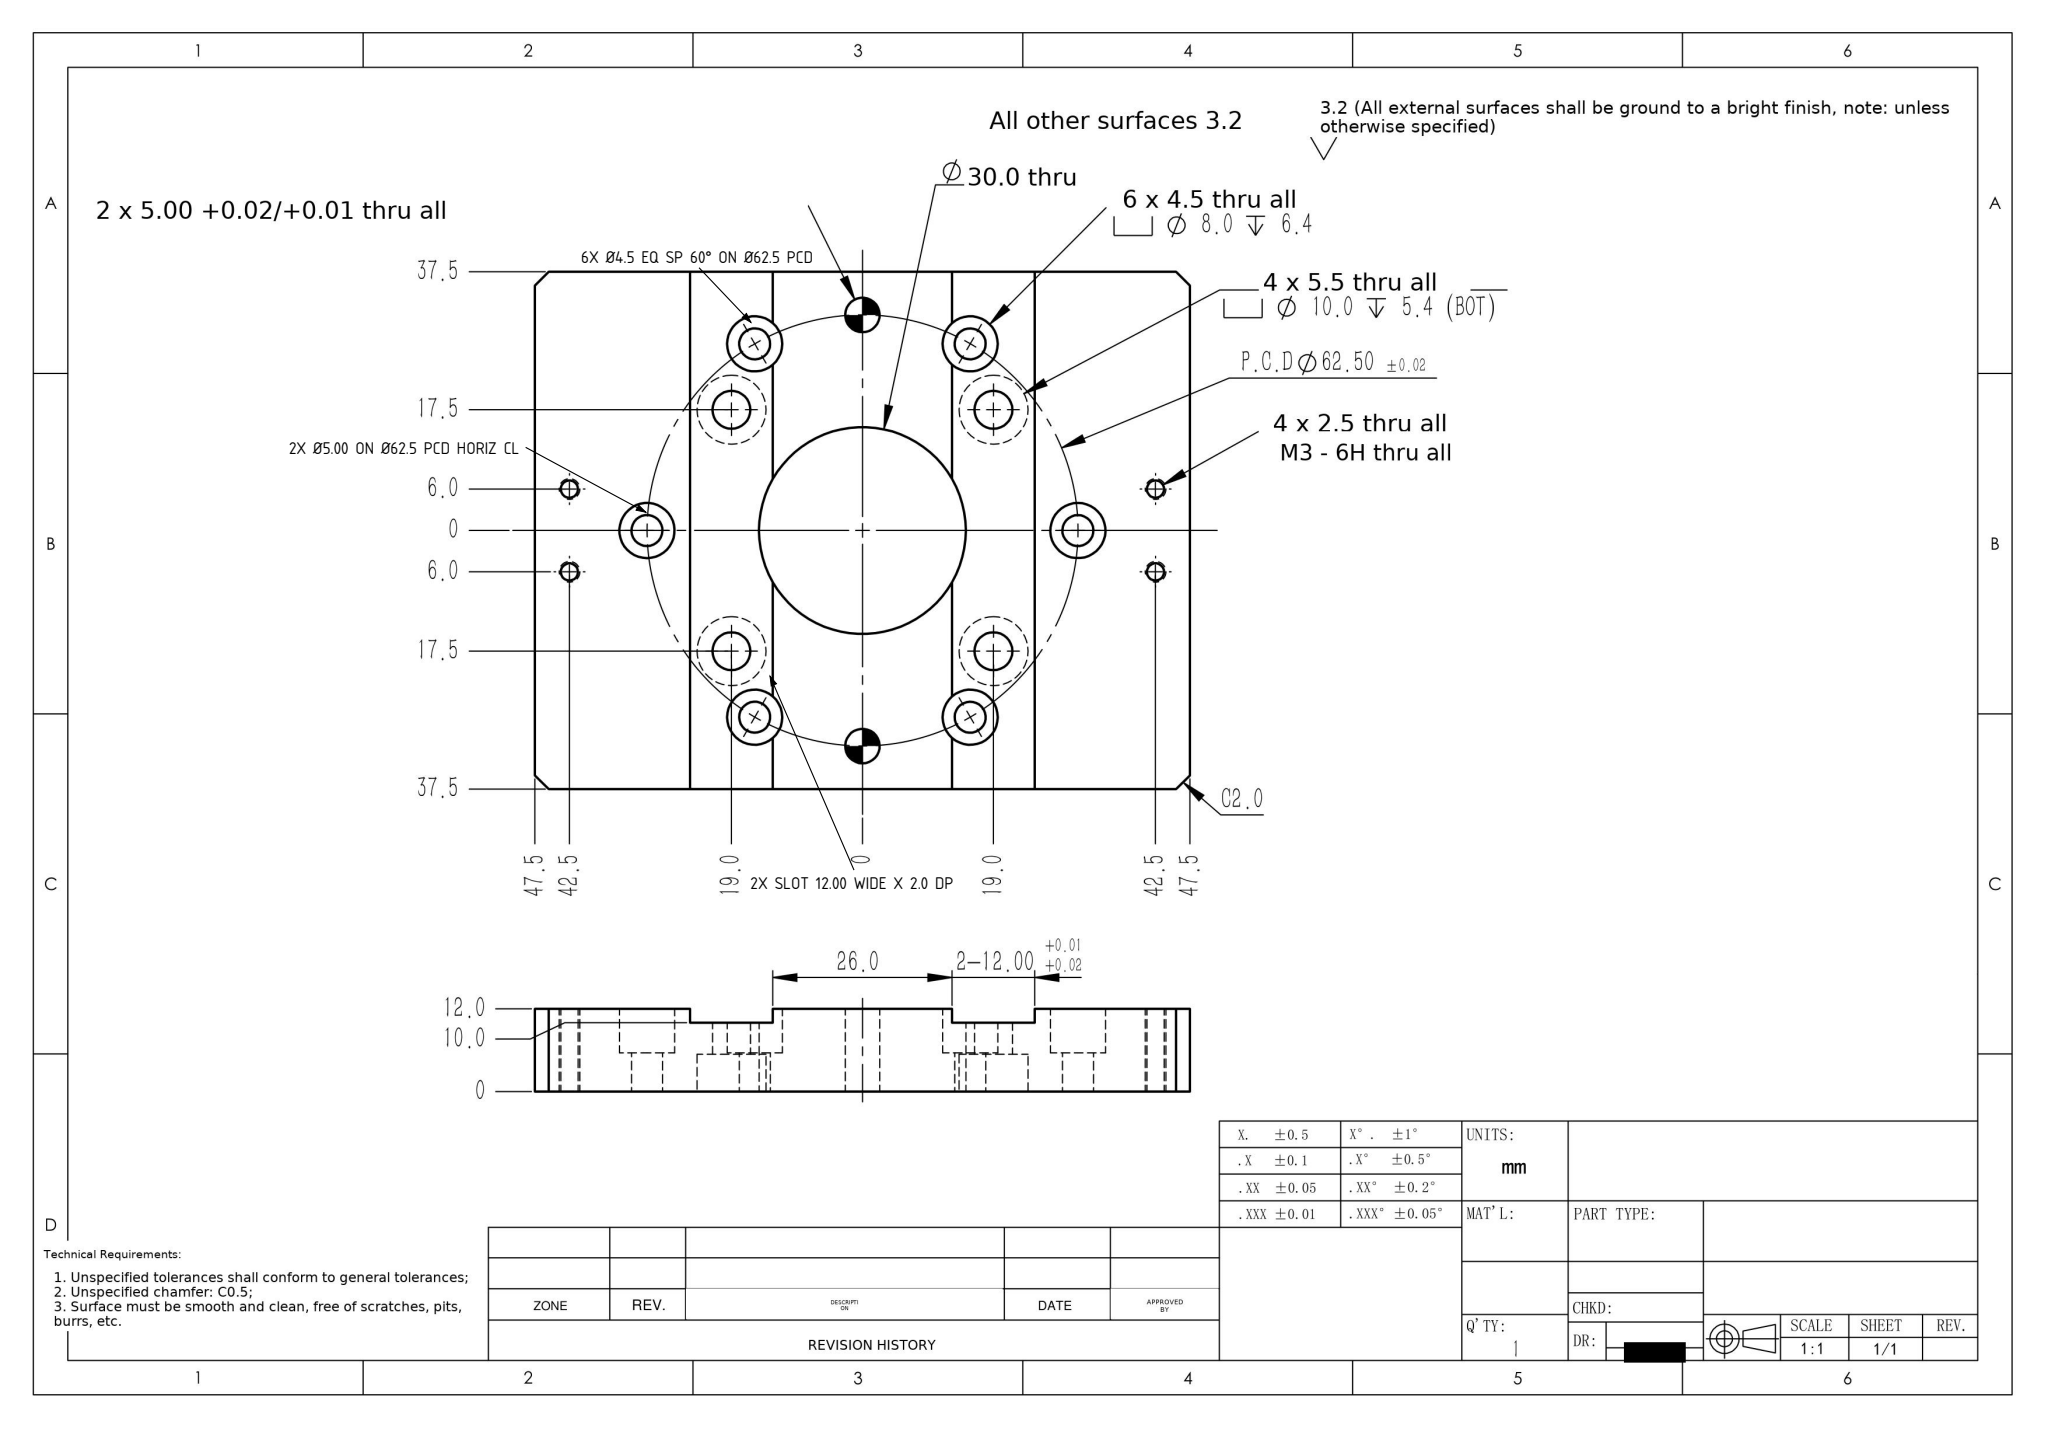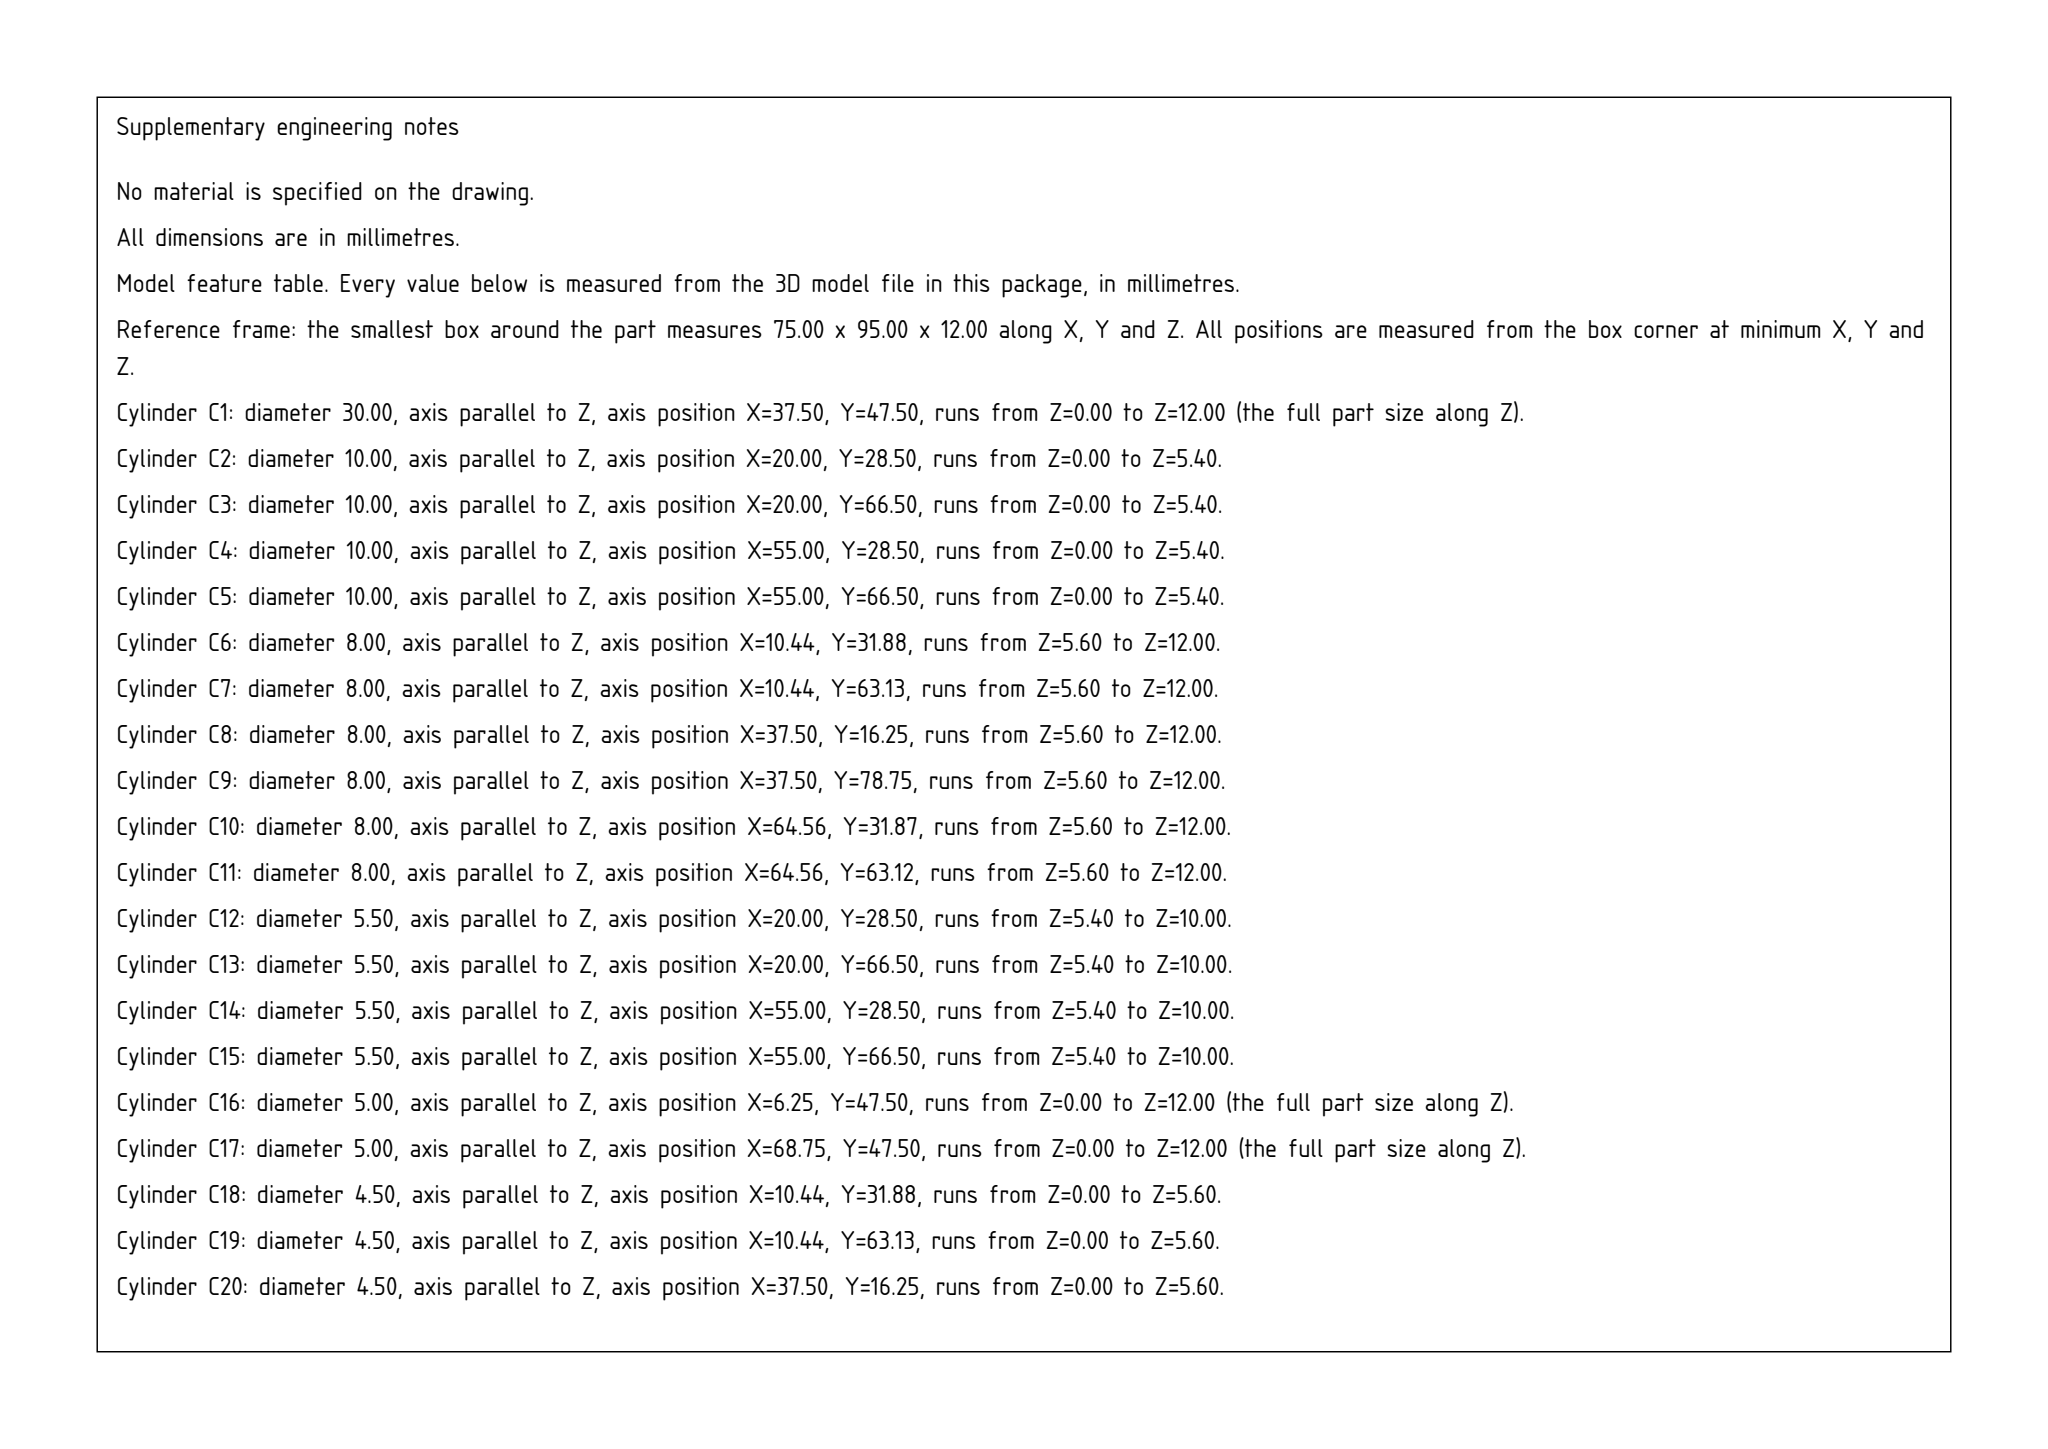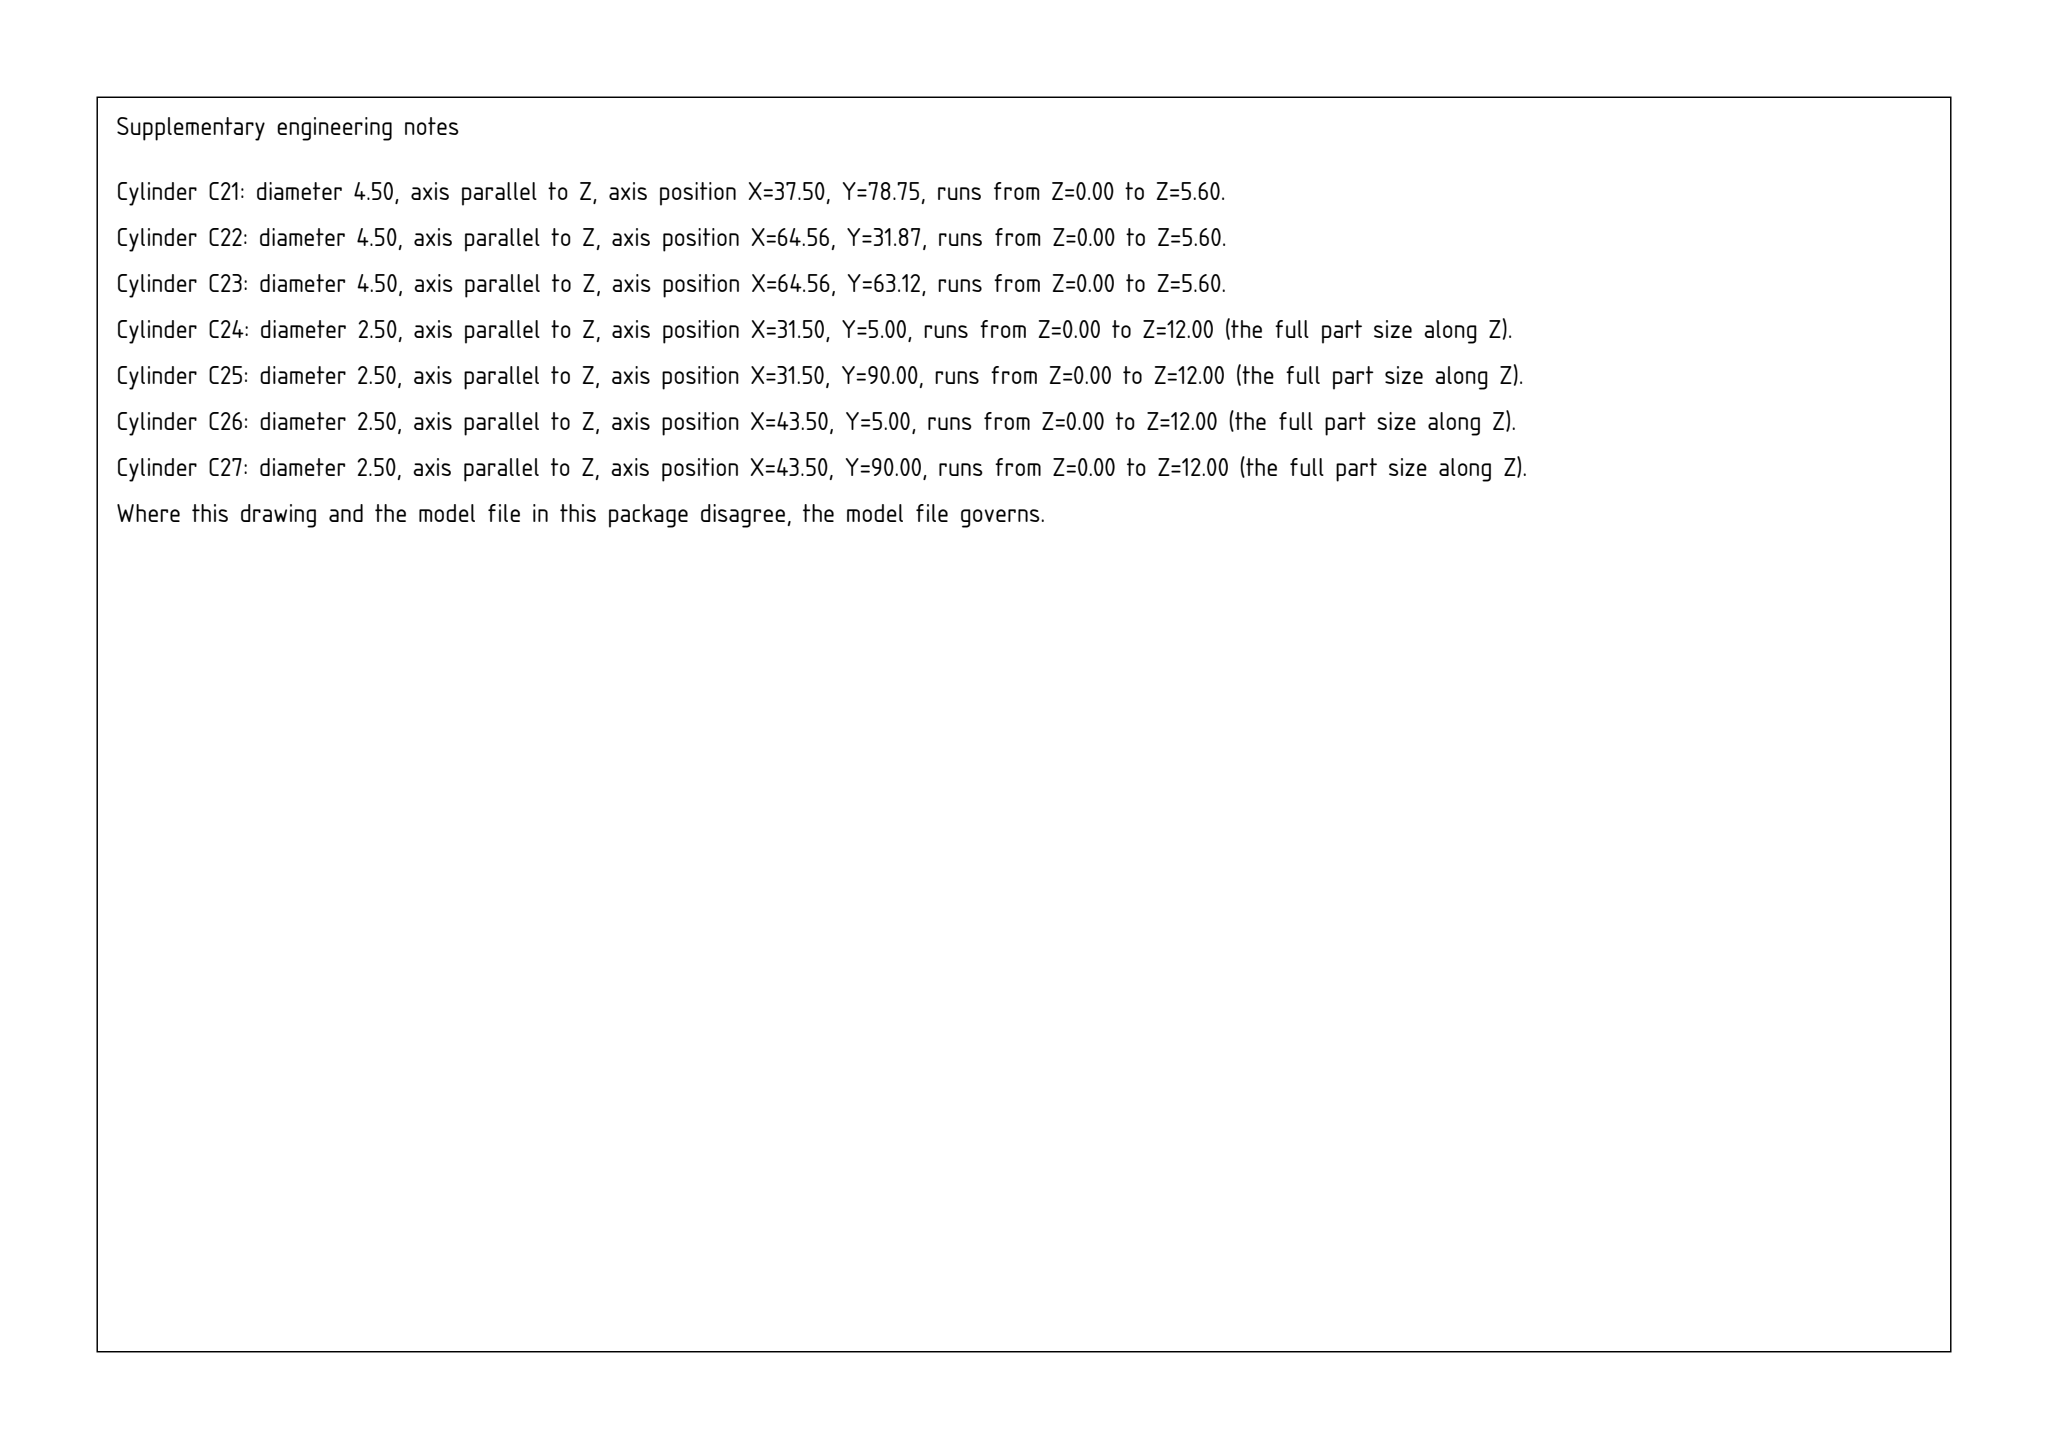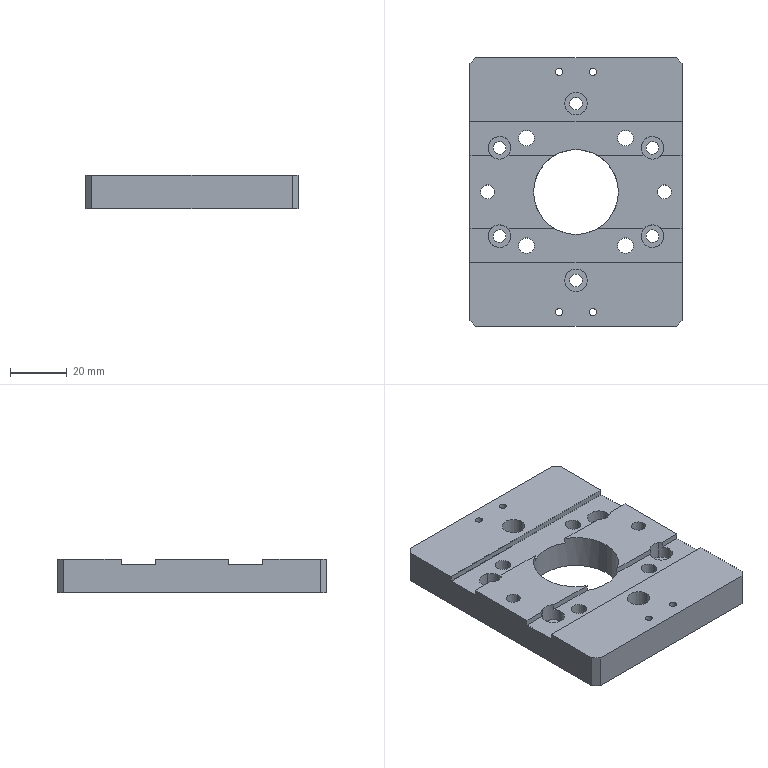Part | SolidWorks | mm | 1 solid | 89 faces | box 75 x 95 x 12 mm | volume 68454 mm3 | cylinder 54 | plane 35 | commonest cylinder face diameters 8 x12 4.5 x12 2.5 x8 10 x8 5.5 x8 5 x4 30 x2
Drawing notes:
2X SLOT 12.00 +0.02/+0.01 WIDE X 2.0 DP FROM TOP FACE | from the solid: Planes y=22.5/34.5 and y=60.5/72.5 (12.00 apart), floors z=10.0 vs top z=12.0 -> 2.0 deep, 2 slots
6X Ø4.5 ON Ø62.50 PCD, EQ SP 60 APART, 2 ON VERT CL | from the solid: Ø4.5 holes at (37.5,78.8),(10.4,63.1),(10.4,31.9),(37.5,16.3),(64.6,31.9),(64.6,63.1) about ctr (37.5,47.5): R=31.25, angles 90/150/210/270/330/30
2X Ø5.00 +0.02/+0.01 THRU ALL ON Ø62.50 PCD, ON HORIZ CL | from the solid: Ø5.0 thru holes z 0-12 at (6.25,47.5) and (68.75,47.5) = ctr (37.5,47.5) ±31.25 on Y=0 centreline
build123d program:
from build123d import *

# Parameters (mm, degrees)
SKETCH1_W                                       = 75
SKETCH1_H                                       = 95
SKETCH1_R                                       = 15
BOSS_EXTRUDE1_DEPTH                             = 12
SKETCH2_W                                       = 75
SKETCH2_H                                       = 12
CUT_EXTRUDE1_DEPTH                              = 2
M4_HEX_SOCKET_HEAD_CAP_SCREW_CBORE1_D           = 4.5
M4_HEX_SOCKET_HEAD_CAP_SCREW_CBORE1_CBORE_D     = 8
M4_HEX_SOCKET_HEAD_CAP_SCREW_CBORE1_CBORE_DEPTH = 6.4
CIRPATTERN1_COUNT                               = 6
SIZE_MM_DOWEL_PIN_HOLE1_D                       = 5
M5_HEX_SOCKET_HEAD_CAP_SCREW_CBORE1_D           = 5.5
M5_HEX_SOCKET_HEAD_CAP_SCREW_CBORE1_CBORE_D     = 10
M5_HEX_SOCKET_HEAD_CAP_SCREW_CBORE1_CBORE_DEPTH = 5.4
M3_TAPPED_HOLE1_D                               = 2.5
CHAMFER1_SIZE                                   = 2


with BuildPart() as part:
    # Sketch1 → Boss-Extrude1 (new body)
    with BuildSketch(Plane.XY):
        Rectangle(SKETCH1_W, SKETCH1_H)
        Circle(SKETCH1_R, mode=Mode.SUBTRACT)
    extrude(amount=BOSS_EXTRUDE1_DEPTH)

    # Sketch2 → Cut-Extrude1 (cut)
    with BuildSketch(Plane.XY.offset(12)):
        with Locations((0, -19)):
            Rectangle(SKETCH2_W, SKETCH2_H)
        with Locations((0, 19)):
            Rectangle(SKETCH2_W, SKETCH2_H)
    extrude(amount=-CUT_EXTRUDE1_DEPTH, mode=Mode.SUBTRACT)

    # M4 Hex Socket Head Cap Screw CBORE1 (through all)
    with Locations(Plane.XY.offset(12)):
        with Locations((0, -31.25)):
            m4_hex_socket_head_cap_screw_cbore1 = CounterBoreHole(M4_HEX_SOCKET_HEAD_CAP_SCREW_CBORE1_D / 2, M4_HEX_SOCKET_HEAD_CAP_SCREW_CBORE1_CBORE_D / 2, M4_HEX_SOCKET_HEAD_CAP_SCREW_CBORE1_CBORE_DEPTH)

    # CirPattern1: M4 Hex Socket Head Cap Screw CBORE1 ×6 about axis
    cirpattern1_axis = Axis((0, 0, 0), (0, 0, 1))
    for i in range(1, CIRPATTERN1_COUNT):
        add(m4_hex_socket_head_cap_screw_cbore1.rotate(cirpattern1_axis, i * 360 / CIRPATTERN1_COUNT), mode=Mode.SUBTRACT)

    # Size mm Dowel Pin Hole1 (through all)
    with Locations(Plane.XY.offset(12)):
        with Locations((31.25, 0), (-31.25, 0)):
            Hole(SIZE_MM_DOWEL_PIN_HOLE1_D / 2)

    # M5 Hex Socket Head Cap Screw CBORE1 (through all)
    with Locations(Plane(origin=(0, 0, 0), x_dir=(1, 0, 0), z_dir=(0, 0, -1))):
        with Locations((17.5, 19), (-17.5, 19), (17.5, -19), (-17.5, -19)):
            CounterBoreHole(M5_HEX_SOCKET_HEAD_CAP_SCREW_CBORE1_D / 2, M5_HEX_SOCKET_HEAD_CAP_SCREW_CBORE1_CBORE_D / 2, M5_HEX_SOCKET_HEAD_CAP_SCREW_CBORE1_CBORE_DEPTH)

    # M3 Tapped Hole1 (through all)
    with Locations(Plane.XY.offset(12)):
        with Locations((-6, -42.5), (6, -42.5), (6, 42.5), (-6, 42.5)):
            Hole(M3_TAPPED_HOLE1_D / 2)

    # Chamfer1
    chamfer1_edges = [part.edges().sort_by_distance(p)[0] for p in [
        (37.5, -47.5, 6),
        (-37.5, -47.5, 6),
        (-37.5, 47.5, 6),
        (37.5, 47.5, 6),
    ]]
    chamfer(chamfer1_edges, length=CHAMFER1_SIZE)


solid = part.part